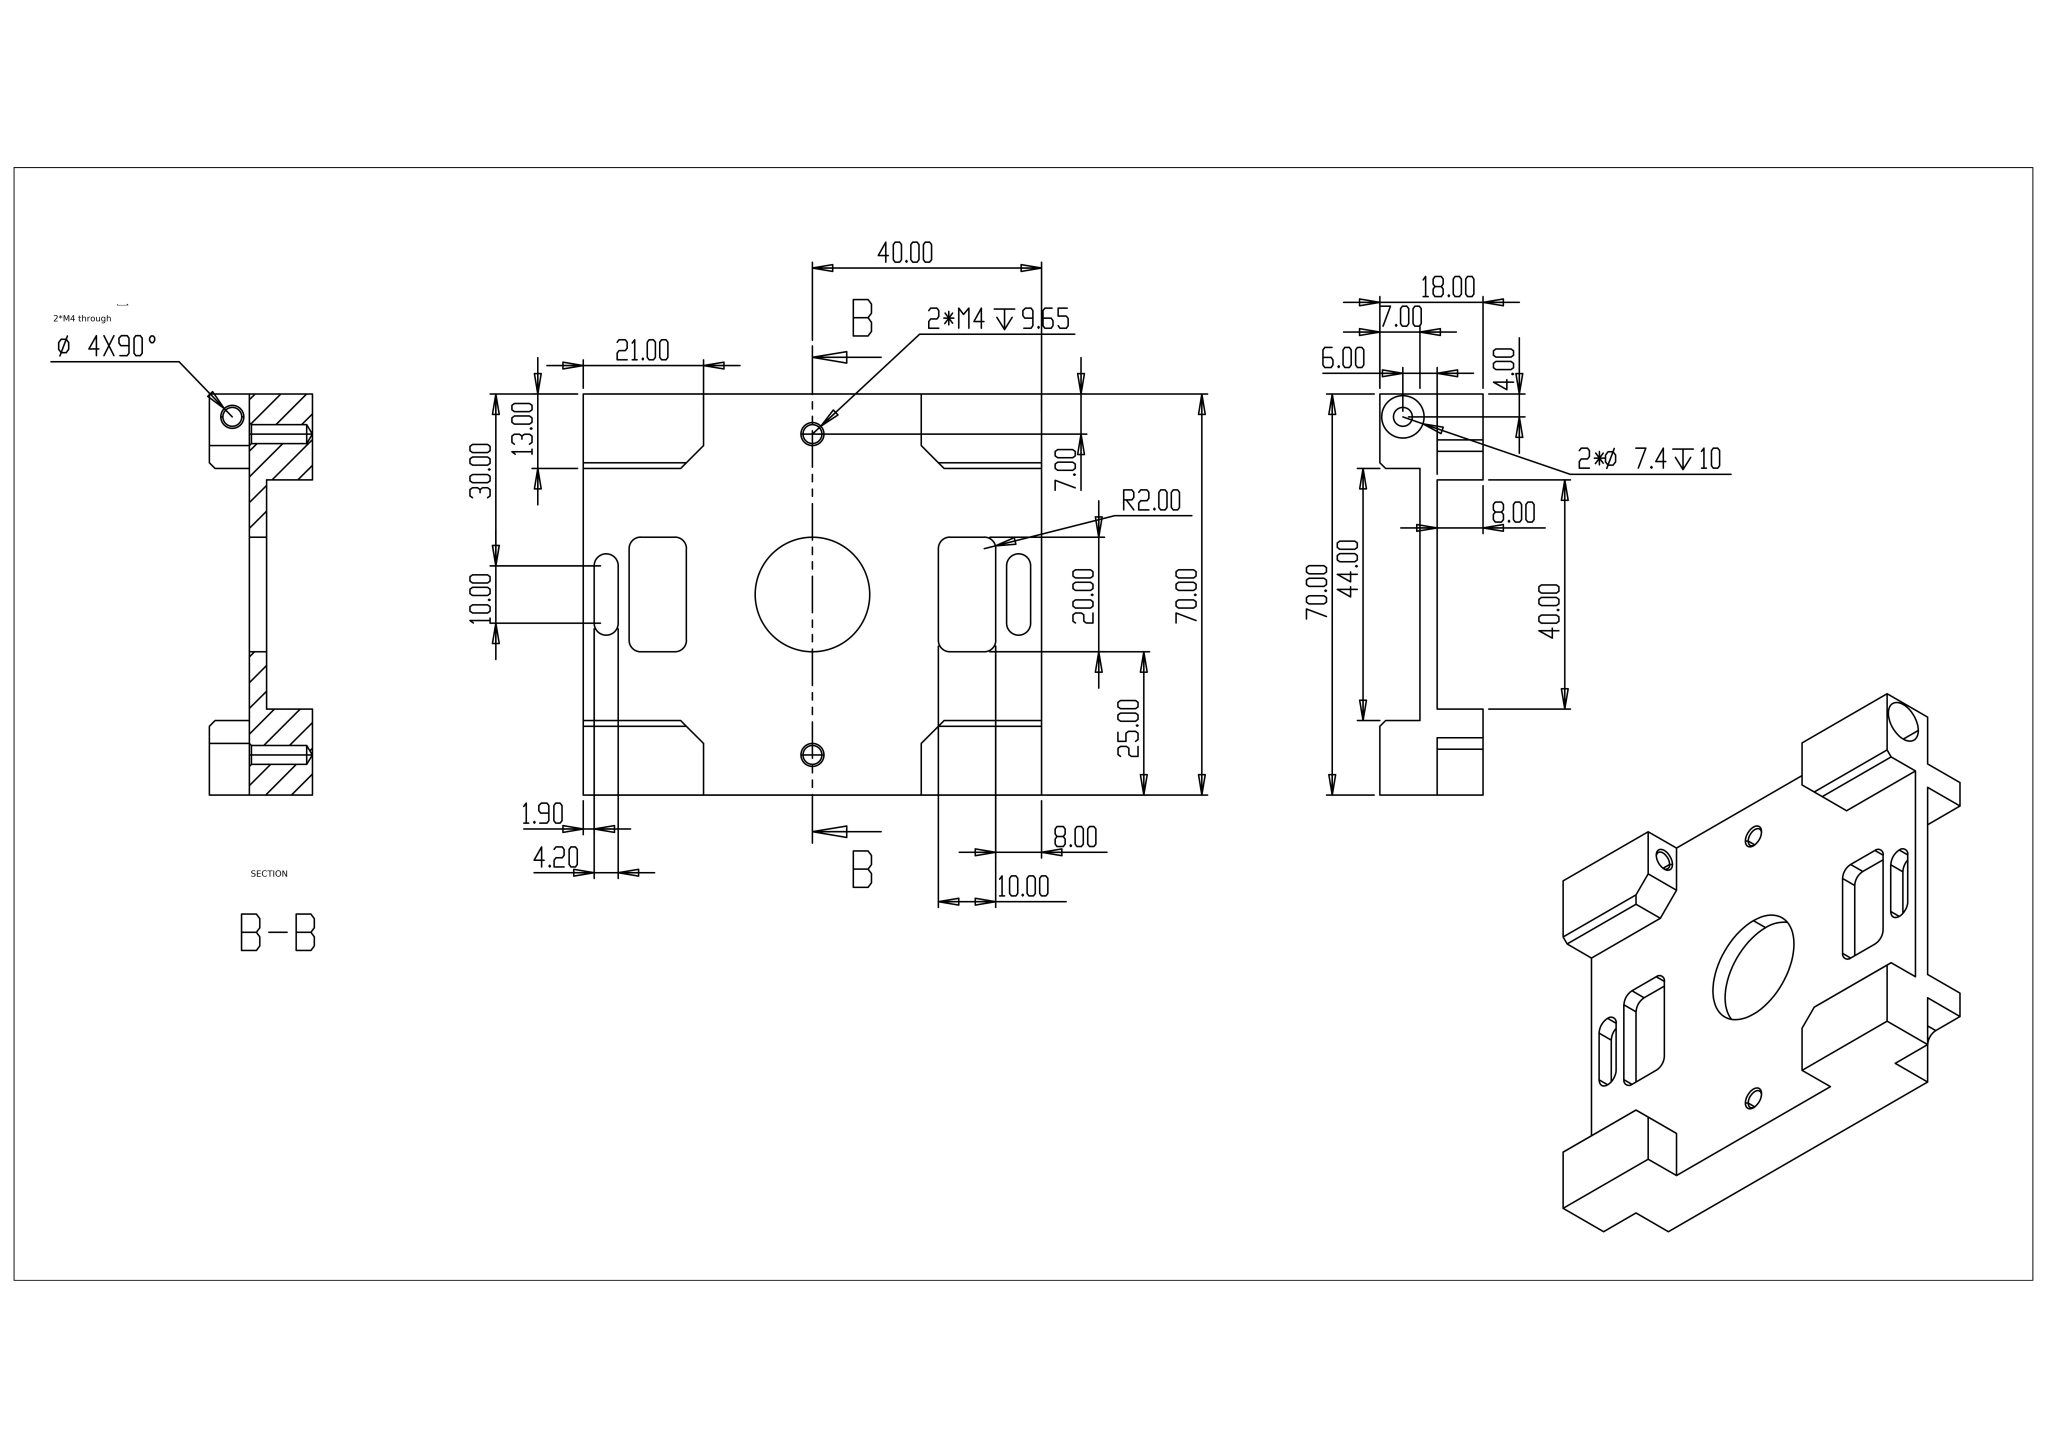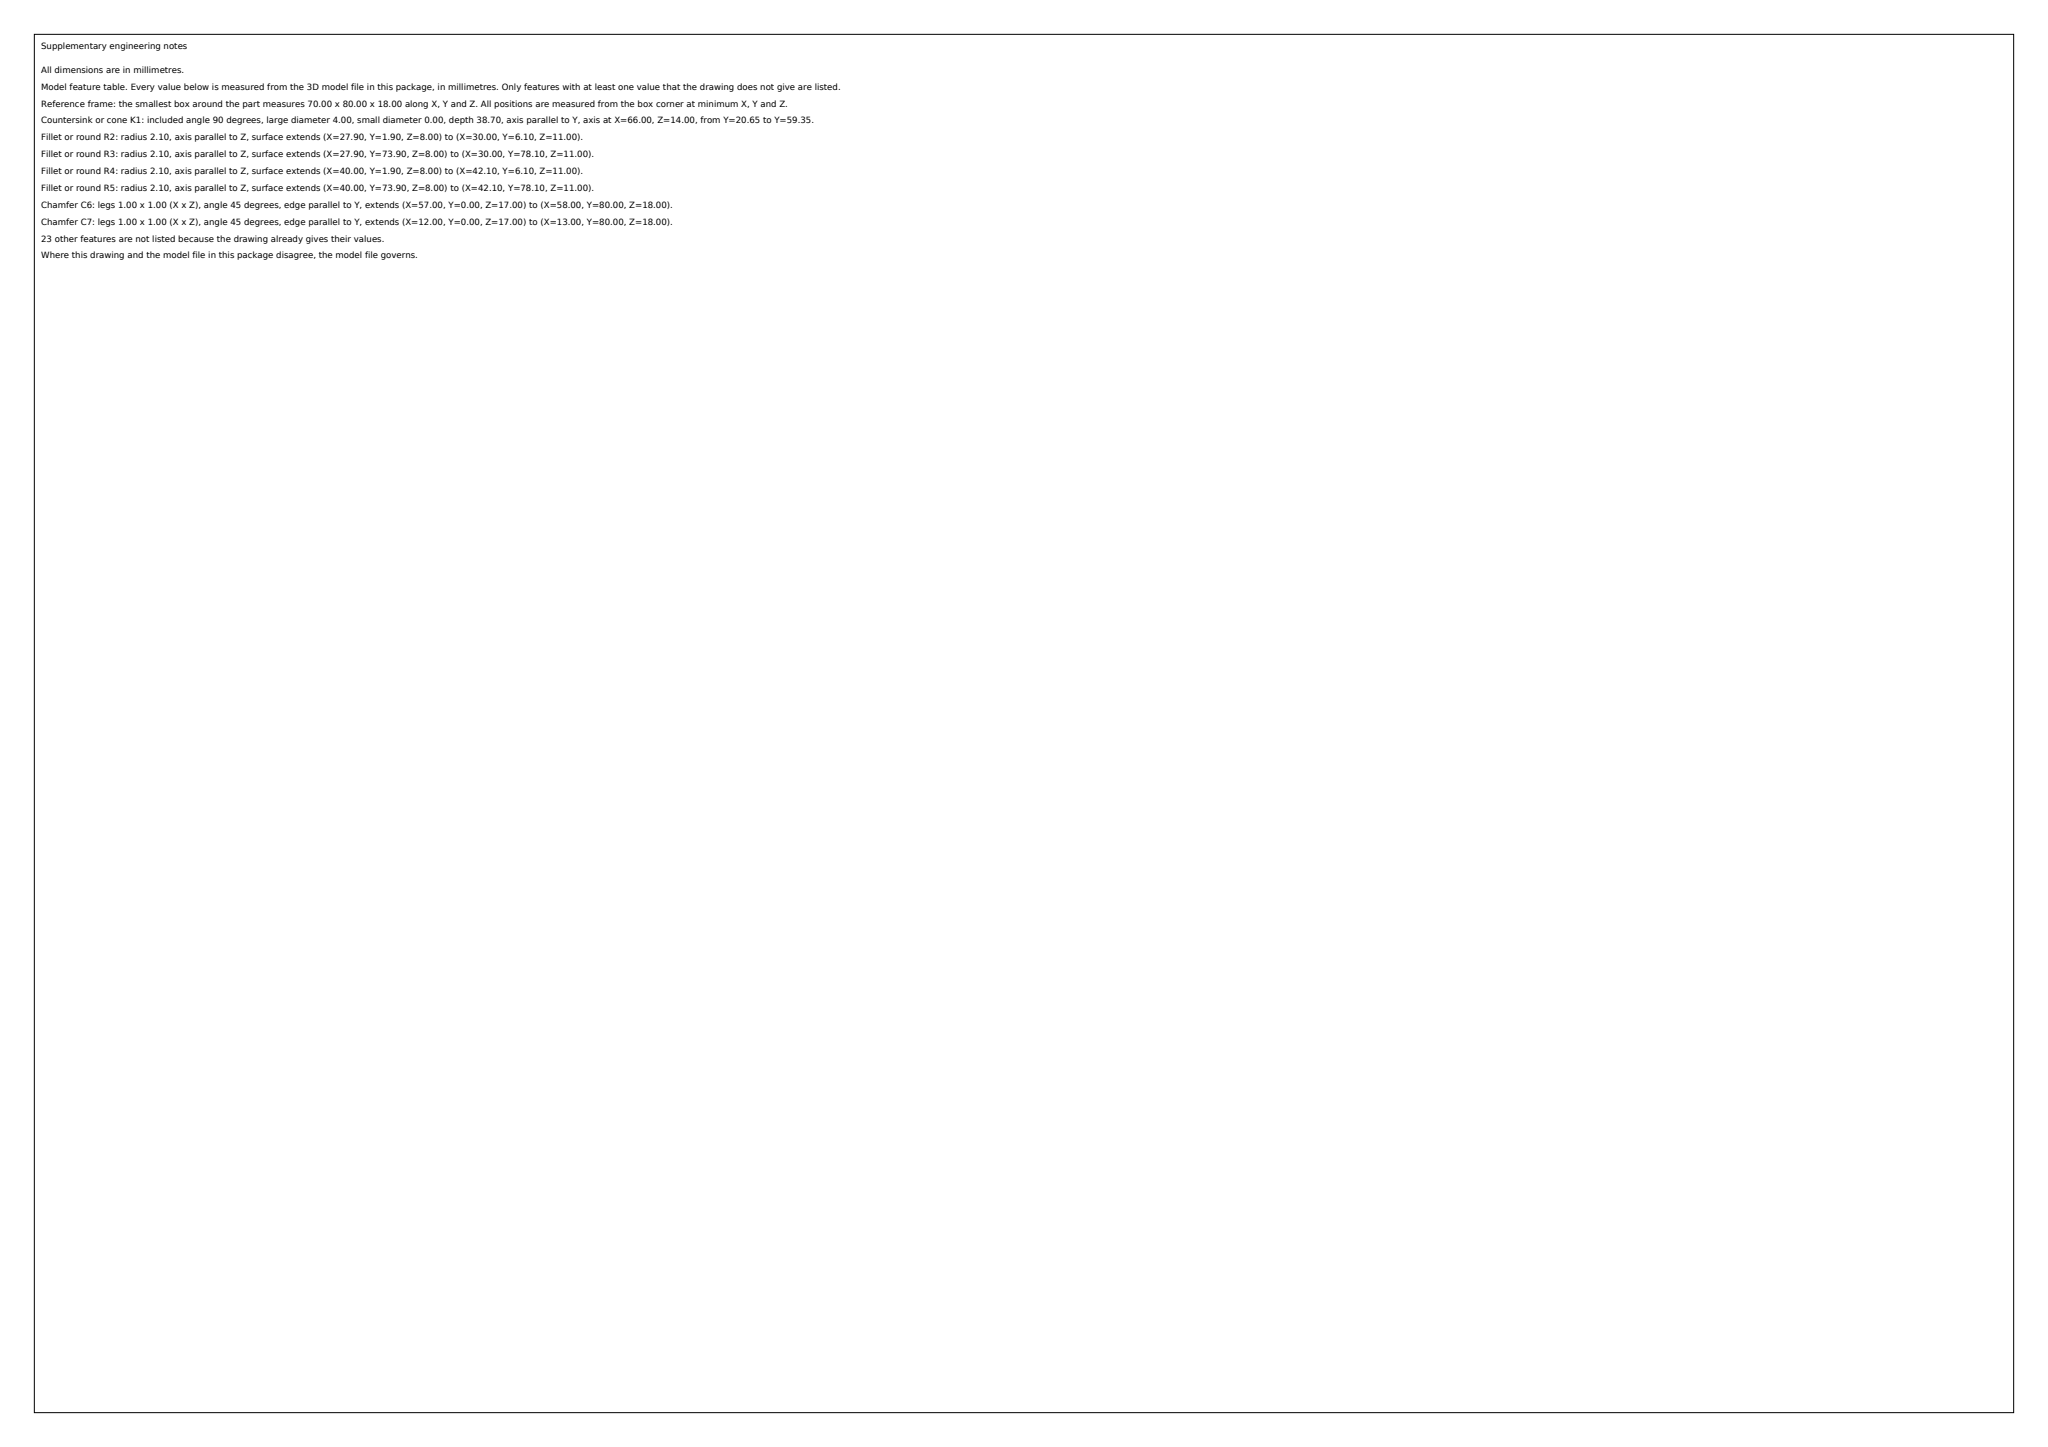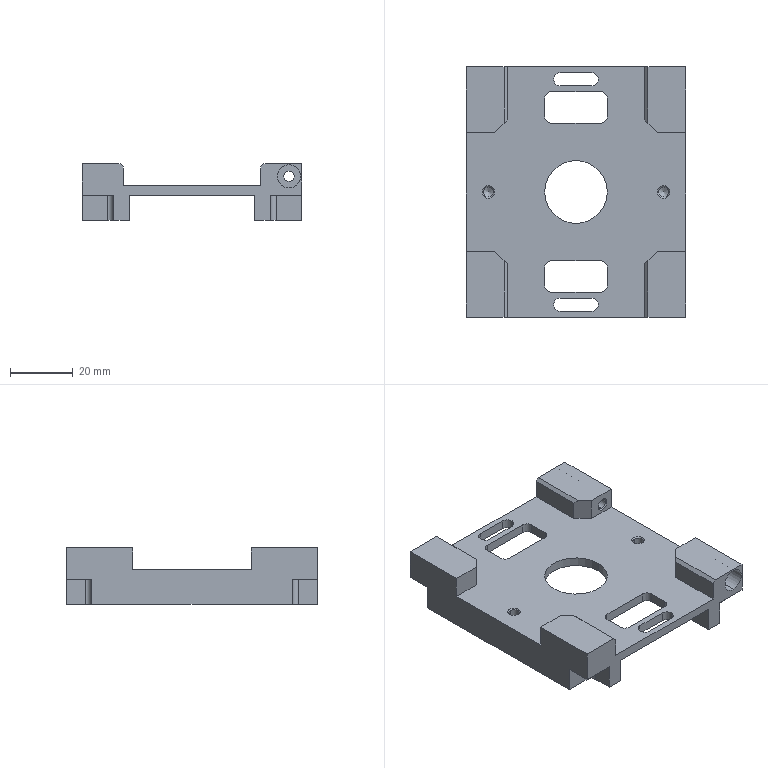Part | SolidWorks | mm | 1 solid | 100 faces | box 70 x 80 x 18 mm | volume 37168 mm3 | plane 56 | cylinder 32 | cone 12 | commonest cylinder face diameters 4 x12 3.3 x8 4.2 x6 7.4 x4 20 x2